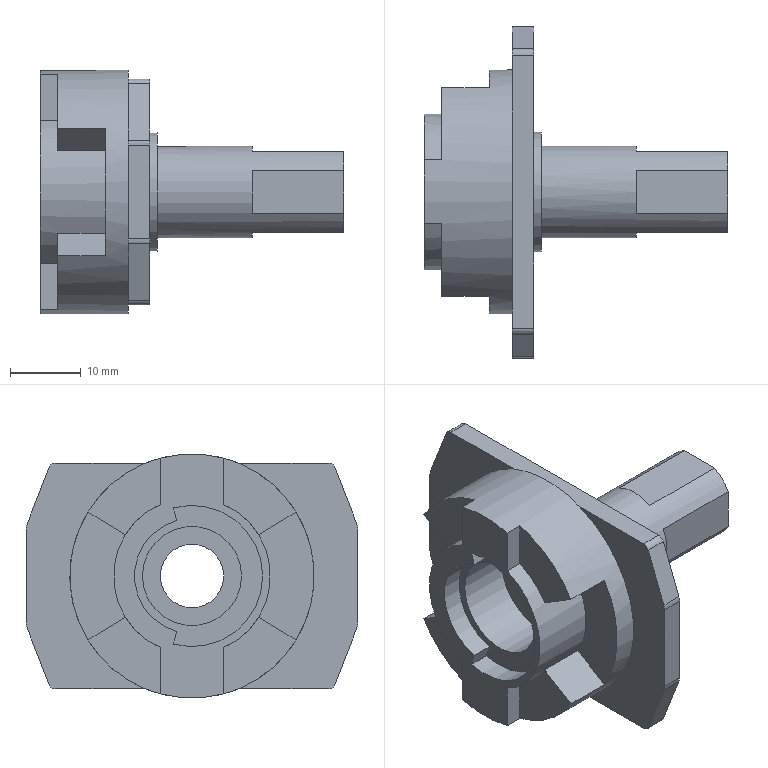Component | NX | CONNECTING_BLOCK | 1 solid | 59 faces | volume 13222 mm3 | plane 42 | cylinder 17 | commonest cylinder face diameters 4 x4 2 x4 22.2 x2 34.6 x1 13 x1 16.9 x1 16.3 x1 20 x1